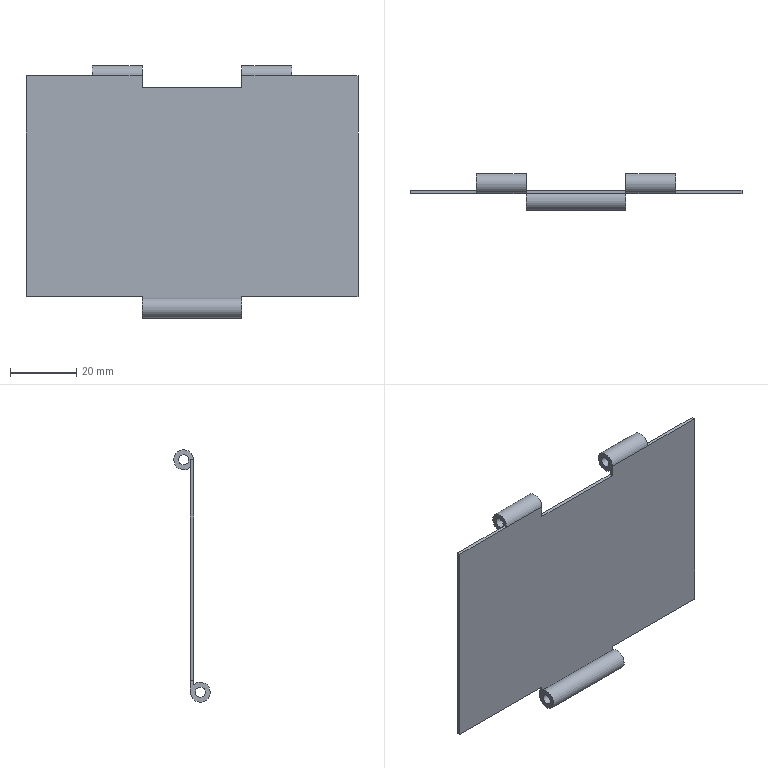Component | NX | PART_2 | 1 solid | 21 faces | volume 7829 mm3 | plane 15 | cylinder 6 | commonest cylinder face diameters 6 x3 3 x3